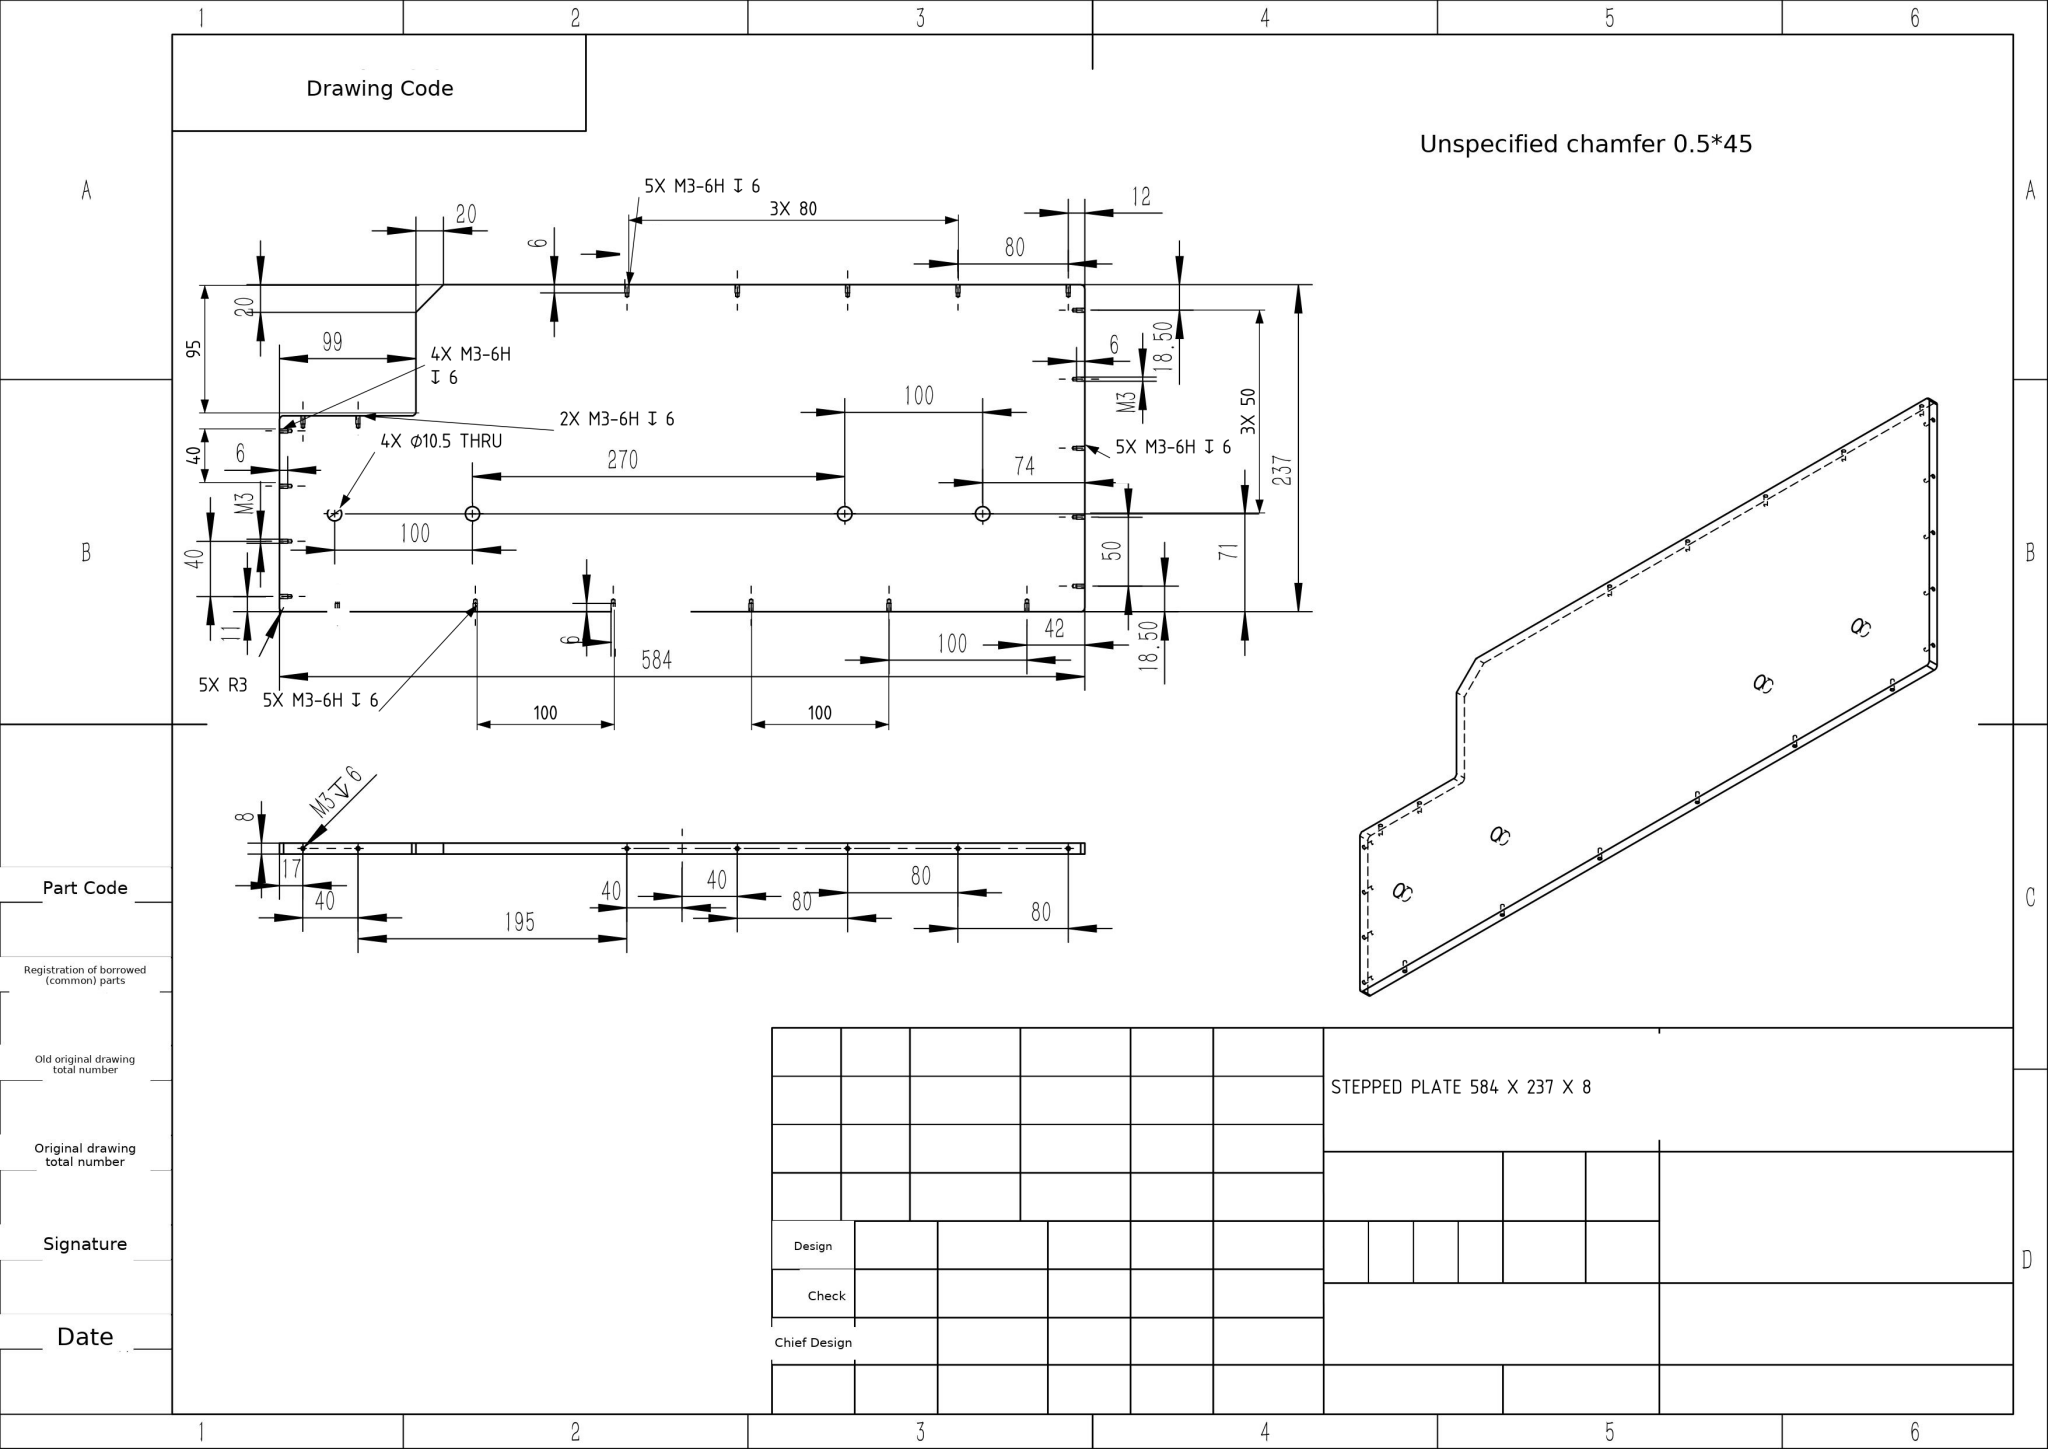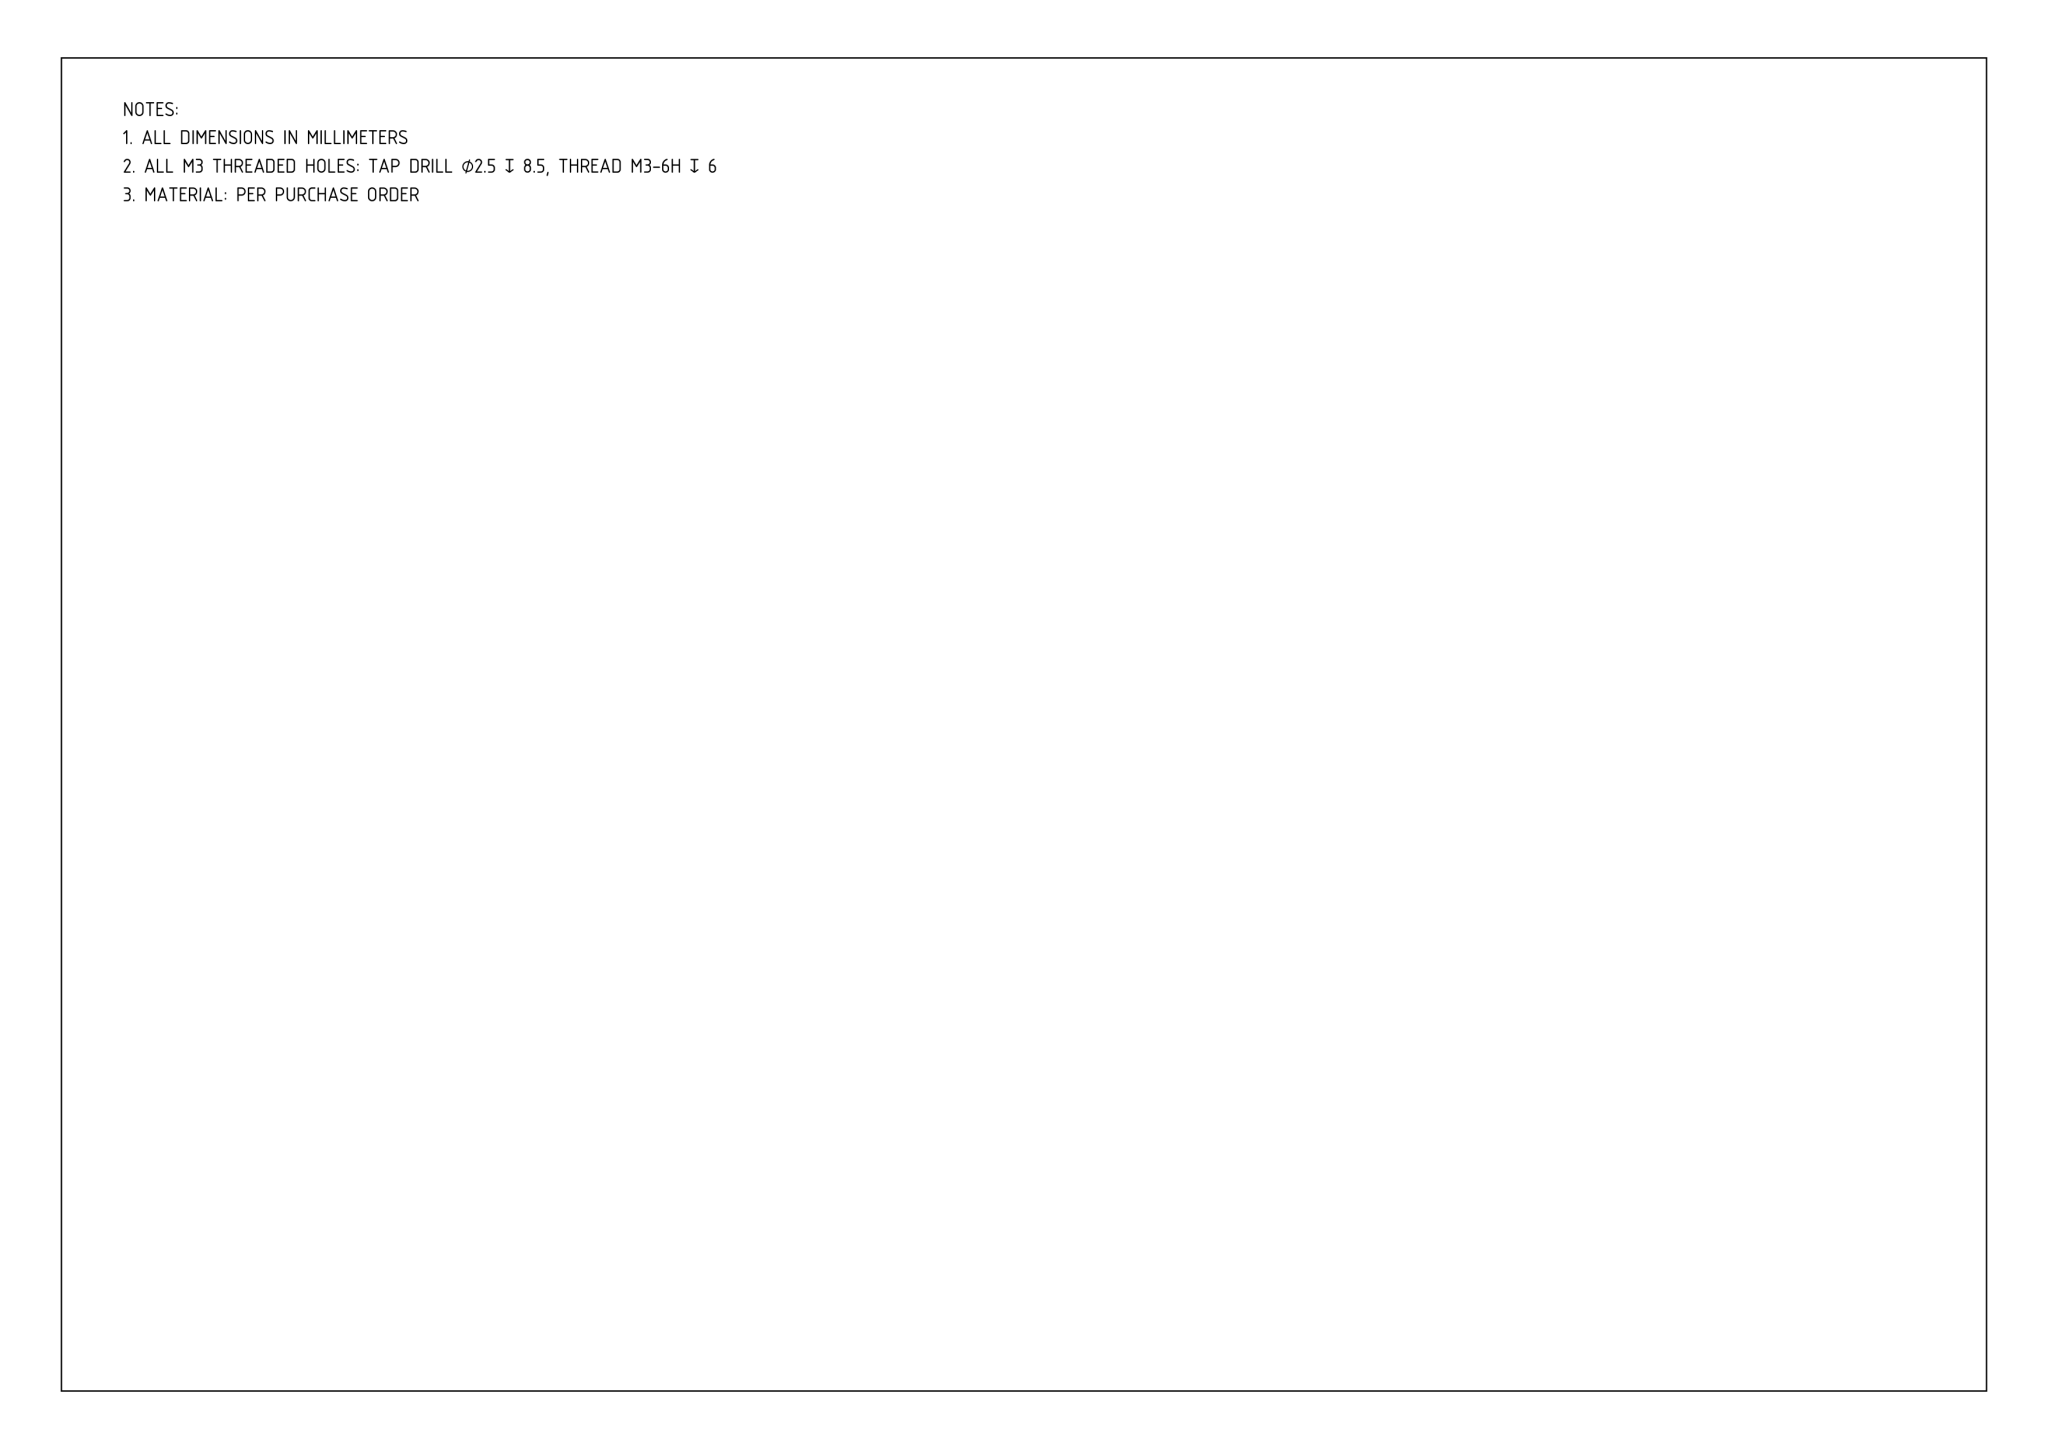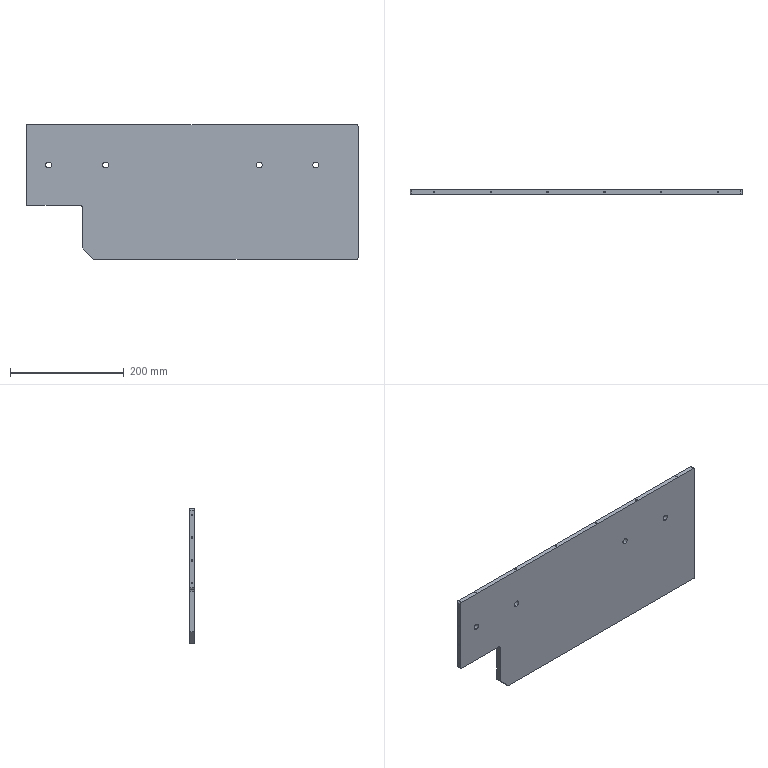Part | NX | mm | 1 solid | 110 faces | box 584 x 8 x 237 mm | volume 1026662 mm3 | cylinder 57 | cone 44 | plane 9 | commonest cylinder face diameters 2.5 x44 10.5 x8 6 x5